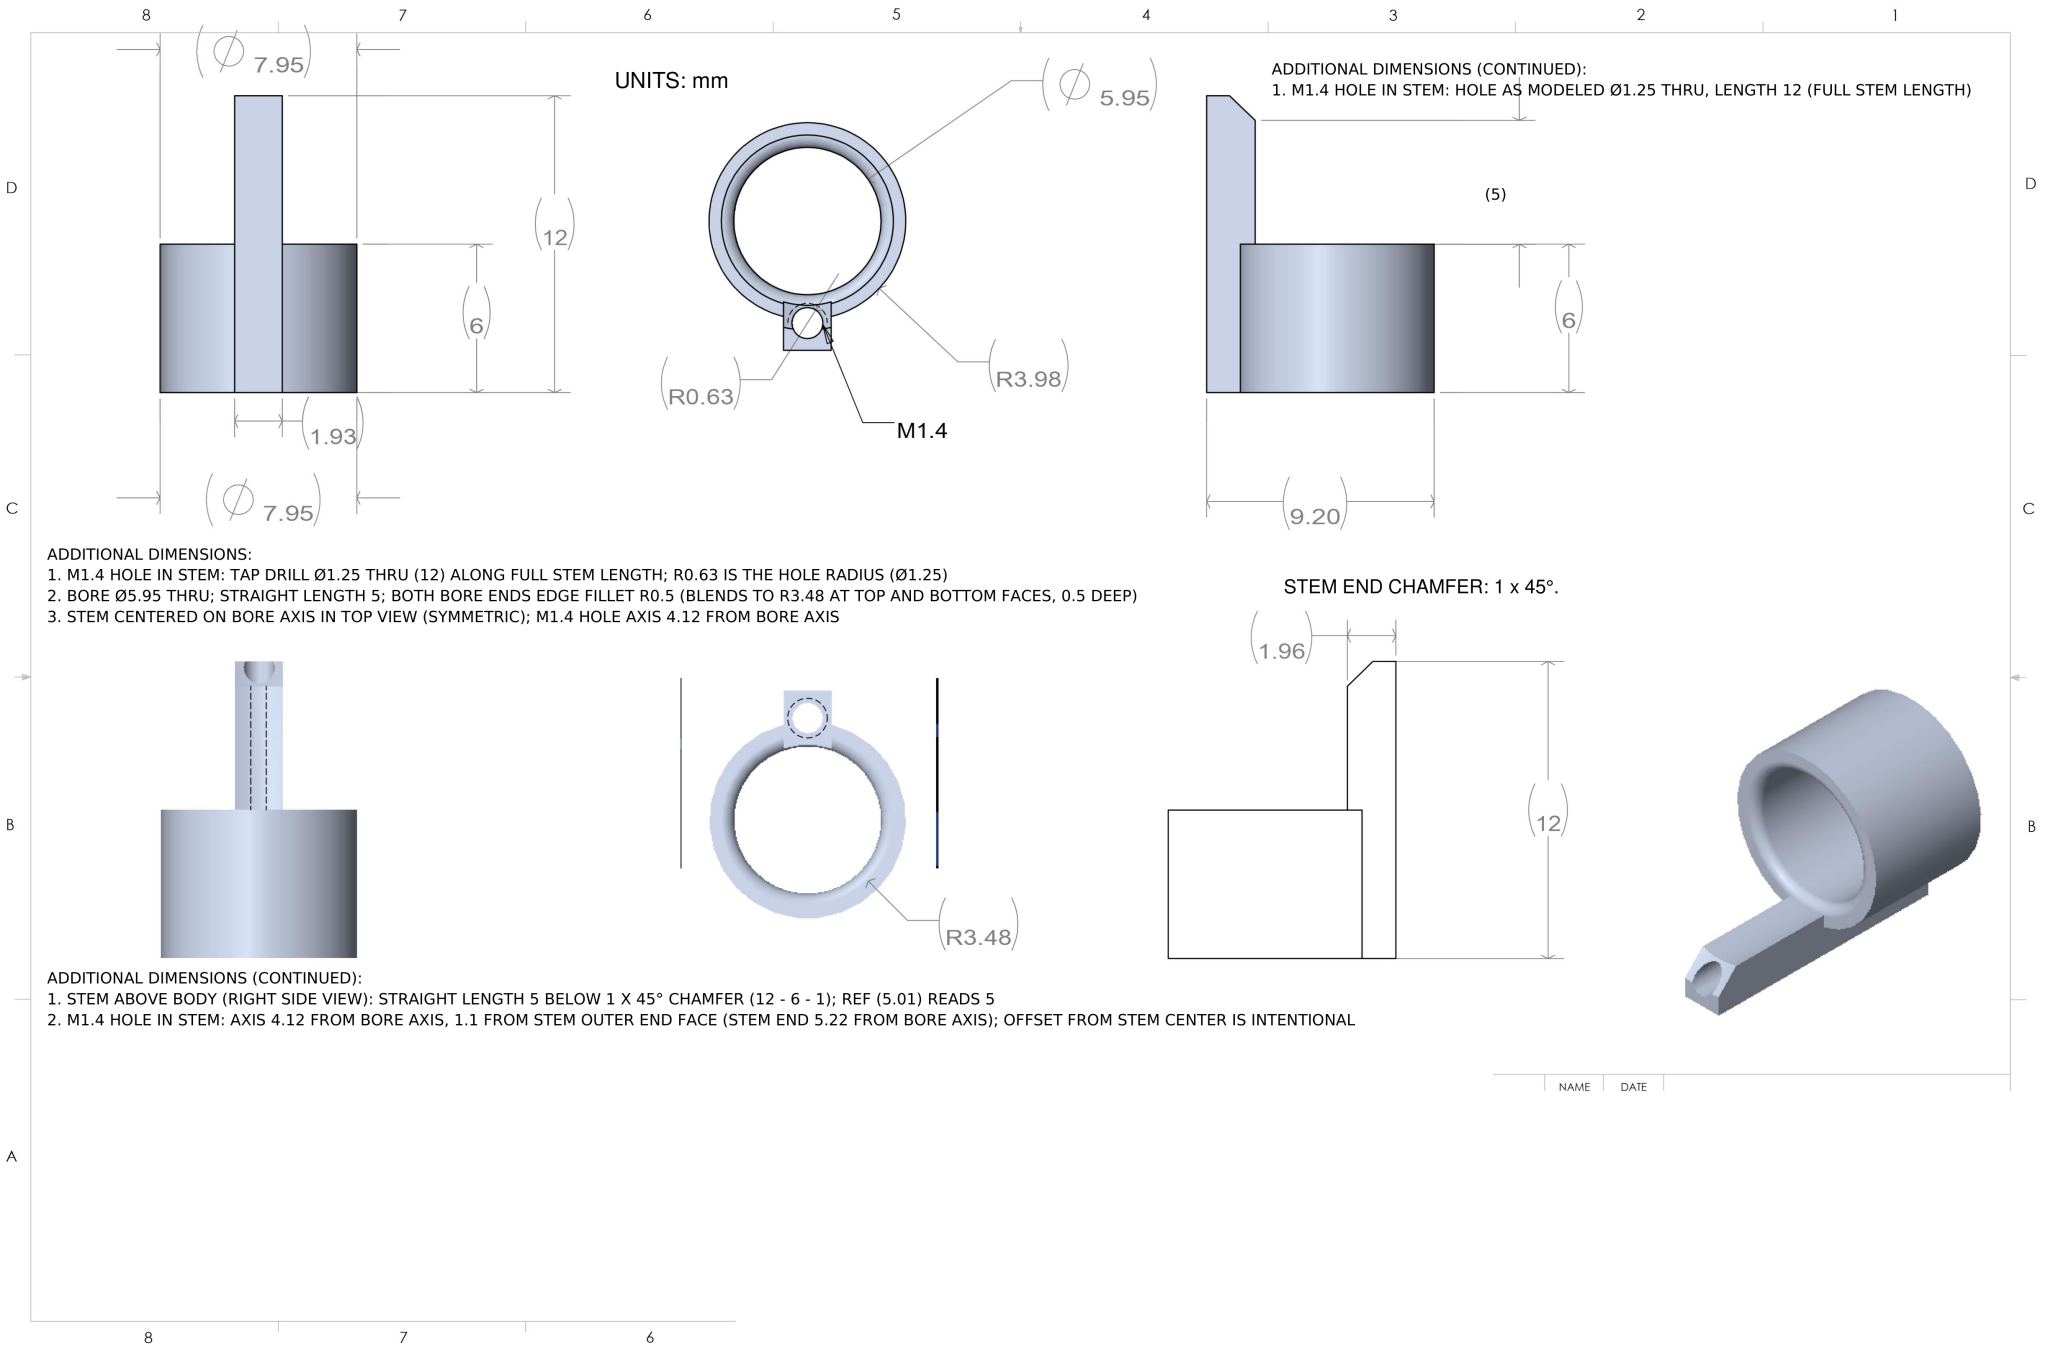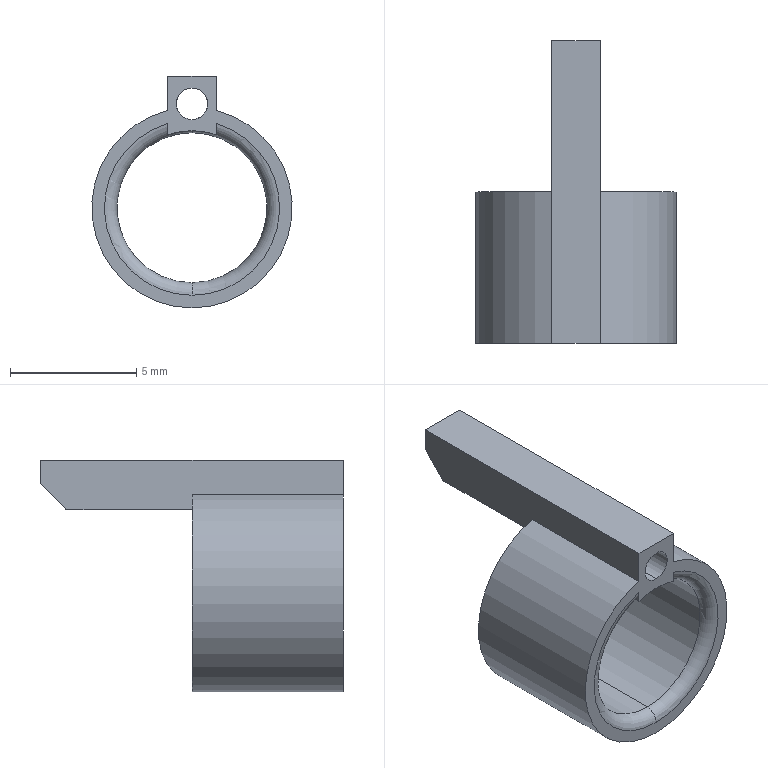Part | NX | mm | 1 solid | 22 faces | box 7.95 x 12 x 9.2 mm | volume 150 mm3 | cylinder 8 | plane 8 | torus 4 | cone 2 | commonest cylinder face diameters 1.25 x2 6.1 x2 5.95 x2 7.95 x1 6.8 x1
STEP:
#1=CARTESIAN_POINT('',(-0.5769,74.,8.153));
#2=VERTEX_POINT('',#1);
#3=CARTESIAN_POINT('',(0.,74.,8.538));
#4=VERTEX_POINT('',#3);
#5=CARTESIAN_POINT('',(0.,74.,7.913));
#6=DIRECTION('',(0.,1.,0.));
#7=DIRECTION('',(0.,0.,1.));
#8=AXIS2_PLACEMENT_3D('',#5,#6,#7);
#9=CIRCLE('',#8,0.625);
#10=EDGE_CURVE('',#2,#4,#9,.T.);
#11=ORIENTED_EDGE('',*,*,#10,.T.);
#12=CARTESIAN_POINT('',(0.,62.,8.538));
#13=VERTEX_POINT('',#12);
#14=CARTESIAN_POINT('',(0.,62.,8.538));
#15=DIRECTION('',(0.,-1.,0.));
#16=VECTOR('',#15,1000.);
#17=LINE('',#14,#16);
#18=EDGE_CURVE('',#4,#13,#17,.T.);
#19=ORIENTED_EDGE('',*,*,#18,.T.);
#20=CARTESIAN_POINT('',(0.,62.,7.288));
#21=VERTEX_POINT('',#20);
#22=CARTESIAN_POINT('',(0.,62.,7.913));
#23=DIRECTION('',(0.,-1.,0.));
#24=DIRECTION('',(0.,0.,-1.));
#25=AXIS2_PLACEMENT_3D('',#22,#23,#24);
#26=CIRCLE('',#25,0.625);
#27=EDGE_CURVE('',#13,#21,#26,.T.);
#28=ORIENTED_EDGE('',*,*,#27,.T.);
#29=CARTESIAN_POINT('',(-0.,73.097,7.288));
#30=VERTEX_POINT('',#29);
#31=CARTESIAN_POINT('',(0.,62.,7.288));
#32=DIRECTION('',(0.,-1.,0.));
#33=VECTOR('',#32,1000.);
#34=LINE('',#31,#33);
#35=EDGE_CURVE('',#30,#21,#34,.T.);
#36=ORIENTED_EDGE('',*,*,#35,.F.);
#37=CARTESIAN_POINT('',(-0.,73.097,7.288));
#38=CARTESIAN_POINT('',(-0.1316,73.097,7.288));
#39=CARTESIAN_POINT('',(-0.2545,73.149,7.332));
#40=CARTESIAN_POINT('',(-0.437,73.287,7.453));
#41=CARTESIAN_POINT('',(-0.5029,73.372,7.53));
#42=CARTESIAN_POINT('',(-0.5938,73.55,7.696));
#43=CARTESIAN_POINT('',(-0.6186,73.641,7.785));
#44=CARTESIAN_POINT('',(-0.6293,73.824,7.968));
#45=CARTESIAN_POINT('',(-0.6149,73.915,8.062));
#46=CARTESIAN_POINT('',(-0.5769,74.,8.153));
#47=B_SPLINE_CURVE_WITH_KNOTS('',3,(#37,#38,#39,#40,#41,#42,#43,#44,#45,#46),.UNSPECIFIED.,.F.,.F.,(4,2,2,2,4),(0.001551,0.001939,0.002327,0.002715,0.003103),.UNSPECIFIED.);
#48=EDGE_CURVE('',#30,#2,#47,.T.);
#49=ORIENTED_EDGE('',*,*,#48,.T.);
#50=EDGE_LOOP('',(#11,#19,#28,#36,#49));
#51=FACE_OUTER_BOUND('',#50,.T.);
#52=CARTESIAN_POINT('',(0.,62.,7.913));
#53=DIRECTION('',(0.,-1.,0.));
#54=DIRECTION('',(0.,0.,-1.));
#55=AXIS2_PLACEMENT_3D('',#52,#53,#54);
#56=CYLINDRICAL_SURFACE('',#55,0.625);
#57=ADVANCED_FACE('',(#51),#56,.F.);
#58=CARTESIAN_POINT('',(0.,73.,7.191));
#59=VERTEX_POINT('',#58);
#60=CARTESIAN_POINT('',(0.963,73.,7.052));
#61=VERTEX_POINT('',#60);
#62=CARTESIAN_POINT('',(0.,73.,3.791));
#63=DIRECTION('',(0.,1.,0.));
#64=DIRECTION('',(0.,0.,1.));
#65=AXIS2_PLACEMENT_3D('',#62,#63,#64);
#66=CIRCLE('',#65,3.4);
#67=EDGE_CURVE('',#59,#61,#66,.T.);
#68=ORIENTED_EDGE('',*,*,#67,.F.);
#69=CARTESIAN_POINT('',(0.,74.,8.191));
#70=DIRECTION('',(0.,0.7071,0.7071));
#71=VECTOR('',#70,1000.);
#72=LINE('',#69,#71);
#73=EDGE_CURVE('',#59,#30,#72,.T.);
#74=ORIENTED_EDGE('',*,*,#73,.T.);
#75=CARTESIAN_POINT('',(0.5769,74.,8.153));
#76=VERTEX_POINT('',#75);
#77=CARTESIAN_POINT('',(0.5769,74.,8.153));
#78=CARTESIAN_POINT('',(0.6149,73.915,8.062));
#79=CARTESIAN_POINT('',(0.6293,73.824,7.968));
#80=CARTESIAN_POINT('',(0.6186,73.642,7.785));
#81=CARTESIAN_POINT('',(0.5936,73.549,7.696));
#82=CARTESIAN_POINT('',(0.5029,73.372,7.53));
#83=CARTESIAN_POINT('',(0.4369,73.287,7.453));
#84=CARTESIAN_POINT('',(0.2542,73.148,7.332));
#85=CARTESIAN_POINT('',(0.1316,73.097,7.288));
#86=CARTESIAN_POINT('',(-0.,73.097,7.288));
#87=B_SPLINE_CURVE_WITH_KNOTS('',3,(#77,#78,#79,#80,#81,#82,#83,#84,#85,#86),.UNSPECIFIED.,.F.,.F.,(4,2,2,2,4),(0.0000003,0.0003881,0.0007758,0.001164,0.001551),.UNSPECIFIED.);
#88=EDGE_CURVE('',#76,#30,#87,.T.);
#89=ORIENTED_EDGE('',*,*,#88,.F.);
#90=CARTESIAN_POINT('',(0.963,74.,8.085));
#91=VERTEX_POINT('',#90);
#92=CARTESIAN_POINT('',(0.,74.,3.791));
#93=DIRECTION('',(0.,-1.,0.));
#94=DIRECTION('',(-0.,0.,1.));
#95=AXIS2_PLACEMENT_3D('',#92,#93,#94);
#96=CIRCLE('',#95,4.4);
#97=EDGE_CURVE('',#91,#76,#96,.T.);
#98=ORIENTED_EDGE('',*,*,#97,.F.);
#99=CARTESIAN_POINT('',(0.963,73.,7.052));
#100=CARTESIAN_POINT('',(0.963,73.332,7.398));
#101=CARTESIAN_POINT('',(0.963,73.665,7.742));
#102=CARTESIAN_POINT('',(0.963,74.,8.085));
#103=B_SPLINE_CURVE_WITH_KNOTS('',3,(#99,#100,#101,#102),.UNSPECIFIED.,.F.,.F.,(4,4),(0.,0.001437),.UNSPECIFIED.);
#104=EDGE_CURVE('',#61,#91,#103,.T.);
#105=ORIENTED_EDGE('',*,*,#104,.F.);
#106=EDGE_LOOP('',(#68,#74,#89,#98,#105));
#107=FACE_OUTER_BOUND('',#106,.T.);
#108=CARTESIAN_POINT('',(0.,74.,3.791));
#109=DIRECTION('',(0.,1.,0.));
#110=DIRECTION('',(0.,0.,1.));
#111=AXIS2_PLACEMENT_3D('',#108,#109,#110);
#112=CONICAL_SURFACE('',#111,4.4,0.7854);
#113=ADVANCED_FACE('',(#107),#112,.F.);
#114=CARTESIAN_POINT('',(0.,68.,0.3163));
#115=VERTEX_POINT('',#114);
#116=CARTESIAN_POINT('',(0.963,68.,7.13));
#117=VERTEX_POINT('',#116);
#118=CARTESIAN_POINT('',(0.,68.,3.791));
#119=DIRECTION('',(0.,-1.,0.));
#120=DIRECTION('',(0.,0.,1.));
#121=AXIS2_PLACEMENT_3D('',#118,#119,#120);
#122=CIRCLE('',#121,3.475);
#123=EDGE_CURVE('',#115,#117,#122,.T.);
#124=ORIENTED_EDGE('',*,*,#123,.F.);
#125=CARTESIAN_POINT('',(0.,67.5,0.8163));
#126=VERTEX_POINT('',#125);
#127=CARTESIAN_POINT('',(0.,67.5,0.3163));
#128=DIRECTION('',(1.,0.,0.));
#129=DIRECTION('',(0.,0.,-1.));
#130=AXIS2_PLACEMENT_3D('',#127,#128,#129);
#131=CIRCLE('',#130,0.5);
#132=EDGE_CURVE('',#115,#126,#131,.T.);
#133=ORIENTED_EDGE('',*,*,#132,.T.);
#134=CARTESIAN_POINT('',(0.,67.5,6.766));
#135=VERTEX_POINT('',#134);
#136=CARTESIAN_POINT('',(0.,67.5,3.791));
#137=DIRECTION('',(0.,1.,0.));
#138=DIRECTION('',(0.,0.,1.));
#139=AXIS2_PLACEMENT_3D('',#136,#137,#138);
#140=CIRCLE('',#139,2.975);
#141=EDGE_CURVE('',#135,#126,#140,.T.);
#142=ORIENTED_EDGE('',*,*,#141,.F.);
#143=CARTESIAN_POINT('',(0.,67.994,7.191));
#144=VERTEX_POINT('',#143);
#145=CARTESIAN_POINT('',(0.,67.5,7.266));
#146=DIRECTION('',(-1.,0.,0.));
#147=DIRECTION('',(0.,0.,1.));
#148=AXIS2_PLACEMENT_3D('',#145,#146,#147);
#149=CIRCLE('',#148,0.5);
#150=EDGE_CURVE('',#144,#135,#149,.T.);
#151=ORIENTED_EDGE('',*,*,#150,.F.);
#152=CARTESIAN_POINT('',(0.963,67.994,7.052));
#153=VERTEX_POINT('',#152);
#154=CARTESIAN_POINT('',(0.,67.994,3.791));
#155=DIRECTION('',(0.,-1.,0.));
#156=DIRECTION('',(0.,0.,-1.));
#157=AXIS2_PLACEMENT_3D('',#154,#155,#156);
#158=CIRCLE('',#157,3.4);
#159=EDGE_CURVE('',#153,#144,#158,.T.);
#160=ORIENTED_EDGE('',*,*,#159,.F.);
#161=CARTESIAN_POINT('',(0.963,67.994,7.052));
#162=CARTESIAN_POINT('',(0.963,67.996,7.065));
#163=CARTESIAN_POINT('',(0.963,67.999,7.091));
#164=CARTESIAN_POINT('',(0.963,68.,7.117));
#165=CARTESIAN_POINT('',(0.963,68.,7.13));
#166=B_SPLINE_CURVE_WITH_KNOTS('',3,(#161,#162,#163,#164,#165),.UNSPECIFIED.,.F.,.F.,(4,1,4),(0.0003591,0.0003981,0.0004371),.UNSPECIFIED.);
#167=EDGE_CURVE('',#153,#117,#166,.T.);
#168=ORIENTED_EDGE('',*,*,#167,.T.);
#169=EDGE_LOOP('',(#124,#133,#142,#151,#160,#168));
#170=FACE_OUTER_BOUND('',#169,.T.);
#171=CARTESIAN_POINT('',(0.,67.5,3.791));
#172=DIRECTION('',(0.,1.,0.));
#173=DIRECTION('',(0.,0.,1.));
#174=AXIS2_PLACEMENT_3D('',#171,#172,#173);
#175=TOROIDAL_SURFACE('',#174,3.475,0.5);
#176=ADVANCED_FACE('',(#170),#175,.T.);
#177=CARTESIAN_POINT('',(0.,62.,6.841));
#178=VERTEX_POINT('',#177);
#179=CARTESIAN_POINT('',(0.963,62.,6.685));
#180=VERTEX_POINT('',#179);
#181=CARTESIAN_POINT('',(0.,62.,3.791));
#182=DIRECTION('',(0.,1.,-0.));
#183=DIRECTION('',(0.,0.,-1.));
#184=AXIS2_PLACEMENT_3D('',#181,#182,#183);
#185=CIRCLE('',#184,3.05);
#186=EDGE_CURVE('',#178,#180,#185,.T.);
#187=ORIENTED_EDGE('',*,*,#186,.F.);
#188=CARTESIAN_POINT('',(0.,62.237,6.841));
#189=VERTEX_POINT('',#188);
#190=CARTESIAN_POINT('',(0.,10.423,6.841));
#191=DIRECTION('',(0.,1.,0.));
#192=VECTOR('',#191,1000.);
#193=LINE('',#190,#192);
#194=EDGE_CURVE('',#178,#189,#193,.T.);
#195=ORIENTED_EDGE('',*,*,#194,.T.);
#196=CARTESIAN_POINT('',(0.963,62.237,6.685));
#197=VERTEX_POINT('',#196);
#198=CARTESIAN_POINT('',(0.,62.237,3.791));
#199=DIRECTION('',(0.,-1.,0.));
#200=DIRECTION('',(0.,0.,1.));
#201=AXIS2_PLACEMENT_3D('',#198,#199,#200);
#202=CIRCLE('',#201,3.05);
#203=EDGE_CURVE('',#197,#189,#202,.T.);
#204=ORIENTED_EDGE('',*,*,#203,.F.);
#205=CARTESIAN_POINT('',(0.963,10.423,6.685));
#206=DIRECTION('',(0.,1.,0.));
#207=VECTOR('',#206,1000.);
#208=LINE('',#205,#207);
#209=EDGE_CURVE('',#180,#197,#208,.T.);
#210=ORIENTED_EDGE('',*,*,#209,.F.);
#211=EDGE_LOOP('',(#187,#195,#204,#210));
#212=FACE_OUTER_BOUND('',#211,.T.);
#213=CARTESIAN_POINT('',(0.,10.423,3.791));
#214=DIRECTION('',(0.,1.,0.));
#215=DIRECTION('',(0.,0.,1.));
#216=AXIS2_PLACEMENT_3D('',#213,#214,#215);
#217=CYLINDRICAL_SURFACE('',#216,3.05);
#218=ADVANCED_FACE('',(#212),#217,.F.);
#219=CARTESIAN_POINT('',(0.,62.5,0.8163));
#220=VERTEX_POINT('',#219);
#221=CARTESIAN_POINT('',(0.,62.5,6.766));
#222=VERTEX_POINT('',#221);
#223=CARTESIAN_POINT('',(0.,62.5,3.791));
#224=DIRECTION('',(0.,-1.,0.));
#225=DIRECTION('',(0.,0.,1.));
#226=AXIS2_PLACEMENT_3D('',#223,#224,#225);
#227=CIRCLE('',#226,2.975);
#228=EDGE_CURVE('',#220,#222,#227,.T.);
#229=ORIENTED_EDGE('',*,*,#228,.F.);
#230=CARTESIAN_POINT('',(0.,62.,0.3163));
#231=VERTEX_POINT('',#230);
#232=CARTESIAN_POINT('',(0.,62.5,0.3163));
#233=DIRECTION('',(1.,0.,0.));
#234=DIRECTION('',(0.,0.,-1.));
#235=AXIS2_PLACEMENT_3D('',#232,#233,#234);
#236=CIRCLE('',#235,0.5);
#237=EDGE_CURVE('',#220,#231,#236,.T.);
#238=ORIENTED_EDGE('',*,*,#237,.T.);
#239=CARTESIAN_POINT('',(0.963,62.,7.13));
#240=VERTEX_POINT('',#239);
#241=CARTESIAN_POINT('',(0.,62.,3.791));
#242=DIRECTION('',(0.,1.,0.));
#243=DIRECTION('',(0.,0.,1.));
#244=AXIS2_PLACEMENT_3D('',#241,#242,#243);
#245=CIRCLE('',#244,3.475);
#246=EDGE_CURVE('',#240,#231,#245,.T.);
#247=ORIENTED_EDGE('',*,*,#246,.F.);
#248=CARTESIAN_POINT('',(0.963,62.,7.13));
#249=CARTESIAN_POINT('',(0.963,62.,7.043));
#250=CARTESIAN_POINT('',(0.963,62.021,6.956));
#251=CARTESIAN_POINT('',(0.963,62.103,6.8));
#252=CARTESIAN_POINT('',(0.963,62.163,6.734));
#253=CARTESIAN_POINT('',(0.963,62.237,6.685));
#254=B_SPLINE_CURVE_WITH_KNOTS('',3,(#248,#249,#250,#251,#252,#253),.UNSPECIFIED.,.F.,.F.,(4,2,4),(0.002836,0.003097,0.003358),.UNSPECIFIED.);
#255=EDGE_CURVE('',#240,#197,#254,.T.);
#256=ORIENTED_EDGE('',*,*,#255,.T.);
#257=ORIENTED_EDGE('',*,*,#203,.T.);
#258=CARTESIAN_POINT('',(0.,62.5,7.266));
#259=DIRECTION('',(-1.,0.,0.));
#260=DIRECTION('',(0.,0.,1.));
#261=AXIS2_PLACEMENT_3D('',#258,#259,#260);
#262=CIRCLE('',#261,0.5);
#263=EDGE_CURVE('',#222,#189,#262,.T.);
#264=ORIENTED_EDGE('',*,*,#263,.F.);
#265=EDGE_LOOP('',(#229,#238,#247,#256,#257,#264));
#266=FACE_OUTER_BOUND('',#265,.T.);
#267=CARTESIAN_POINT('',(0.,62.5,3.791));
#268=DIRECTION('',(0.,1.,0.));
#269=DIRECTION('',(0.,0.,1.));
#270=AXIS2_PLACEMENT_3D('',#267,#268,#269);
#271=TOROIDAL_SURFACE('',#270,3.475,0.5);
#272=ADVANCED_FACE('',(#266),#271,.T.);
#273=CARTESIAN_POINT('',(0.,62.5,3.791));
#274=DIRECTION('',(0.,-1.,0.));
#275=DIRECTION('',(0.,0.,1.));
#276=AXIS2_PLACEMENT_3D('',#273,#274,#275);
#277=CIRCLE('',#276,2.975);
#278=EDGE_CURVE('',#222,#220,#277,.T.);
#279=ORIENTED_EDGE('',*,*,#278,.T.);
#280=CARTESIAN_POINT('',(0.,62.,0.8163));
#281=DIRECTION('',(0.,1.,0.));
#282=VECTOR('',#281,1000.);
#283=LINE('',#280,#282);
#284=EDGE_CURVE('',#220,#126,#283,.T.);
#285=ORIENTED_EDGE('',*,*,#284,.T.);
#286=CARTESIAN_POINT('',(0.,67.5,3.791));
#287=DIRECTION('',(0.,1.,0.));
#288=DIRECTION('',(0.,0.,1.));
#289=AXIS2_PLACEMENT_3D('',#286,#287,#288);
#290=CIRCLE('',#289,2.975);
#291=EDGE_CURVE('',#126,#135,#290,.T.);
#292=ORIENTED_EDGE('',*,*,#291,.T.);
#293=CARTESIAN_POINT('',(0.,62.,6.766));
#294=DIRECTION('',(0.,1.,0.));
#295=VECTOR('',#294,1000.);
#296=LINE('',#293,#295);
#297=EDGE_CURVE('',#222,#135,#296,.T.);
#298=ORIENTED_EDGE('',*,*,#297,.F.);
#299=EDGE_LOOP('',(#279,#285,#292,#298));
#300=FACE_OUTER_BOUND('',#299,.T.);
#301=CARTESIAN_POINT('',(0.,62.,3.791));
#302=DIRECTION('',(0.,1.,0.));
#303=DIRECTION('',(0.,0.,1.));
#304=AXIS2_PLACEMENT_3D('',#301,#302,#303);
#305=CYLINDRICAL_SURFACE('',#304,2.975);
#306=ADVANCED_FACE('',(#300),#305,.F.);
#307=ORIENTED_EDGE('',*,*,#284,.F.);
#308=ORIENTED_EDGE('',*,*,#228,.T.);
#309=ORIENTED_EDGE('',*,*,#297,.T.);
#310=ORIENTED_EDGE('',*,*,#141,.T.);
#311=EDGE_LOOP('',(#307,#308,#309,#310));
#312=FACE_OUTER_BOUND('',#311,.T.);
#313=CARTESIAN_POINT('',(0.,62.,3.791));
#314=DIRECTION('',(0.,1.,0.));
#315=DIRECTION('',(0.,0.,1.));
#316=AXIS2_PLACEMENT_3D('',#313,#314,#315);
#317=CYLINDRICAL_SURFACE('',#316,2.975);
#318=ADVANCED_FACE('',(#312),#317,.F.);
#319=CARTESIAN_POINT('',(0.963,62.,6.38));
#320=DIRECTION('',(0.,0.,1.));
#321=VECTOR('',#320,1000.);
#322=LINE('',#319,#321);
#323=EDGE_CURVE('',#180,#240,#322,.T.);
#324=ORIENTED_EDGE('',*,*,#323,.F.);
#325=ORIENTED_EDGE('',*,*,#209,.T.);
#326=ORIENTED_EDGE('',*,*,#255,.F.);
#327=EDGE_LOOP('',(#324,#325,#326));
#328=FACE_OUTER_BOUND('',#327,.T.);
#329=CARTESIAN_POINT('',(0.963,74.,6.38));
#330=DIRECTION('',(-1.,0.,0.));
#331=DIRECTION('',(0.,0.,1.));
#332=AXIS2_PLACEMENT_3D('',#329,#330,#331);
#333=PLANE('',#332);
#334=ADVANCED_FACE('',(#328),#333,.F.);
#335=ORIENTED_EDGE('',*,*,#237,.F.);
#336=ORIENTED_EDGE('',*,*,#278,.F.);
#337=ORIENTED_EDGE('',*,*,#263,.T.);
#338=CARTESIAN_POINT('',(-0.963,62.237,6.685));
#339=VERTEX_POINT('',#338);
#340=CARTESIAN_POINT('',(0.,62.237,3.791));
#341=DIRECTION('',(0.,-1.,0.));
#342=DIRECTION('',(0.,0.,1.));
#343=AXIS2_PLACEMENT_3D('',#340,#341,#342);
#344=CIRCLE('',#343,3.05);
#345=EDGE_CURVE('',#189,#339,#344,.T.);
#346=ORIENTED_EDGE('',*,*,#345,.T.);
#347=CARTESIAN_POINT('',(-0.963,62.,7.13));
#348=VERTEX_POINT('',#347);
#349=CARTESIAN_POINT('',(-0.963,62.237,6.685));
#350=CARTESIAN_POINT('',(-0.963,62.164,6.733));
#351=CARTESIAN_POINT('',(-0.963,62.103,6.801));
#352=CARTESIAN_POINT('',(-0.963,62.022,6.955));
#353=CARTESIAN_POINT('',(-0.963,62.,7.042));
#354=CARTESIAN_POINT('',(-0.963,62.,7.13));
#355=B_SPLINE_CURVE_WITH_KNOTS('',3,(#349,#350,#351,#352,#353,#354),.UNSPECIFIED.,.F.,.F.,(4,2,4),(0.003024,0.003285,0.003546),.UNSPECIFIED.);
#356=EDGE_CURVE('',#339,#348,#355,.T.);
#357=ORIENTED_EDGE('',*,*,#356,.T.);
#358=CARTESIAN_POINT('',(0.,62.,3.791));
#359=DIRECTION('',(0.,1.,0.));
#360=DIRECTION('',(0.,0.,1.));
#361=AXIS2_PLACEMENT_3D('',#358,#359,#360);
#362=CIRCLE('',#361,3.475);
#363=EDGE_CURVE('',#231,#348,#362,.T.);
#364=ORIENTED_EDGE('',*,*,#363,.F.);
#365=EDGE_LOOP('',(#335,#336,#337,#346,#357,#364));
#366=FACE_OUTER_BOUND('',#365,.T.);
#367=CARTESIAN_POINT('',(0.,62.5,3.791));
#368=DIRECTION('',(0.,1.,0.));
#369=DIRECTION('',(0.,0.,1.));
#370=AXIS2_PLACEMENT_3D('',#367,#368,#369);
#371=TOROIDAL_SURFACE('',#370,3.475,0.5);
#372=ADVANCED_FACE('',(#366),#371,.T.);
#373=CARTESIAN_POINT('',(-0.963,62.,6.685));
#374=VERTEX_POINT('',#373);
#375=CARTESIAN_POINT('',(-0.963,62.,6.38));
#376=DIRECTION('',(-0.,-0.,-1.));
#377=VECTOR('',#376,1000.);
#378=LINE('',#375,#377);
#379=EDGE_CURVE('',#348,#374,#378,.T.);
#380=ORIENTED_EDGE('',*,*,#379,.F.);
#381=ORIENTED_EDGE('',*,*,#356,.F.);
#382=CARTESIAN_POINT('',(-0.963,10.423,6.685));
#383=DIRECTION('',(0.,-1.,0.));
#384=VECTOR('',#383,1000.);
#385=LINE('',#382,#384);
#386=EDGE_CURVE('',#339,#374,#385,.T.);
#387=ORIENTED_EDGE('',*,*,#386,.T.);
#388=EDGE_LOOP('',(#380,#381,#387));
#389=FACE_OUTER_BOUND('',#388,.T.);
#390=CARTESIAN_POINT('',(-0.963,74.,6.38));
#391=DIRECTION('',(1.,0.,-0.));
#392=DIRECTION('',(-0.,0.,-1.));
#393=AXIS2_PLACEMENT_3D('',#390,#391,#392);
#394=PLANE('',#393);
#395=ADVANCED_FACE('',(#389),#394,.F.);
#396=ORIENTED_EDGE('',*,*,#194,.F.);
#397=CARTESIAN_POINT('',(0.,62.,3.791));
#398=DIRECTION('',(0.,1.,-0.));
#399=DIRECTION('',(0.,0.,-1.));
#400=AXIS2_PLACEMENT_3D('',#397,#398,#399);
#401=CIRCLE('',#400,3.05);
#402=EDGE_CURVE('',#374,#178,#401,.T.);
#403=ORIENTED_EDGE('',*,*,#402,.F.);
#404=ORIENTED_EDGE('',*,*,#386,.F.);
#405=ORIENTED_EDGE('',*,*,#345,.F.);
#406=EDGE_LOOP('',(#396,#403,#404,#405));
#407=FACE_OUTER_BOUND('',#406,.T.);
#408=CARTESIAN_POINT('',(0.,10.423,3.791));
#409=DIRECTION('',(0.,1.,0.));
#410=DIRECTION('',(0.,0.,1.));
#411=AXIS2_PLACEMENT_3D('',#408,#409,#410);
#412=CYLINDRICAL_SURFACE('',#411,3.05);
#413=ADVANCED_FACE('',(#407),#412,.F.);
#414=CARTESIAN_POINT('',(0.963,68.,7.648));
#415=VERTEX_POINT('',#414);
#416=CARTESIAN_POINT('',(-0.963,68.,7.648));
#417=VERTEX_POINT('',#416);
#418=CARTESIAN_POINT('',(0.,68.,3.791));
#419=DIRECTION('',(0.,1.,0.));
#420=DIRECTION('',(1.,0.,0.));
#421=AXIS2_PLACEMENT_3D('',#418,#419,#420);
#422=CIRCLE('',#421,3.975);
#423=EDGE_CURVE('',#415,#417,#422,.T.);
#424=ORIENTED_EDGE('',*,*,#423,.F.);
#425=CARTESIAN_POINT('',(0.963,62.,7.648));
#426=VERTEX_POINT('',#425);
#427=CARTESIAN_POINT('',(0.963,62.,7.648));
#428=DIRECTION('',(0.,-1.,0.));
#429=VECTOR('',#428,1000.);
#430=LINE('',#427,#429);
#431=EDGE_CURVE('',#415,#426,#430,.T.);
#432=ORIENTED_EDGE('',*,*,#431,.T.);
#433=CARTESIAN_POINT('',(-0.963,62.,7.648));
#434=VERTEX_POINT('',#433);
#435=CARTESIAN_POINT('',(0.,62.,3.791));
#436=DIRECTION('',(0.,1.,0.));
#437=DIRECTION('',(1.,0.,0.));
#438=AXIS2_PLACEMENT_3D('',#435,#436,#437);
#439=CIRCLE('',#438,3.975);
#440=EDGE_CURVE('',#426,#434,#439,.T.);
#441=ORIENTED_EDGE('',*,*,#440,.T.);
#442=CARTESIAN_POINT('',(-0.963,62.,7.648));
#443=DIRECTION('',(0.,1.,0.));
#444=VECTOR('',#443,1000.);
#445=LINE('',#442,#444);
#446=EDGE_CURVE('',#434,#417,#445,.T.);
#447=ORIENTED_EDGE('',*,*,#446,.T.);
#448=EDGE_LOOP('',(#424,#432,#441,#447));
#449=FACE_OUTER_BOUND('',#448,.T.);
#450=CARTESIAN_POINT('',(0.,62.,3.791));
#451=DIRECTION('',(0.,1.,0.));
#452=DIRECTION('',(0.,0.,1.));
#453=AXIS2_PLACEMENT_3D('',#450,#451,#452);
#454=CYLINDRICAL_SURFACE('',#453,3.975);
#455=ADVANCED_FACE('',(#449),#454,.T.);
#456=CARTESIAN_POINT('',(-0.963,68.,7.13));
#457=VERTEX_POINT('',#456);
#458=CARTESIAN_POINT('',(0.,68.,3.791));
#459=DIRECTION('',(0.,-1.,0.));
#460=DIRECTION('',(0.,0.,1.));
#461=AXIS2_PLACEMENT_3D('',#458,#459,#460);
#462=CIRCLE('',#461,3.475);
#463=EDGE_CURVE('',#457,#115,#462,.T.);
#464=ORIENTED_EDGE('',*,*,#463,.T.);
#465=ORIENTED_EDGE('',*,*,#123,.T.);
#466=CARTESIAN_POINT('',(0.963,68.,3.791));
#467=DIRECTION('',(0.,0.,1.));
#468=VECTOR('',#467,1000.);
#469=LINE('',#466,#468);
#470=EDGE_CURVE('',#117,#415,#469,.T.);
#471=ORIENTED_EDGE('',*,*,#470,.T.);
#472=ORIENTED_EDGE('',*,*,#423,.T.);
#473=CARTESIAN_POINT('',(-0.963,68.,3.791));
#474=DIRECTION('',(-0.,0.,-1.));
#475=VECTOR('',#474,1000.);
#476=LINE('',#473,#475);
#477=EDGE_CURVE('',#417,#457,#476,.T.);
#478=ORIENTED_EDGE('',*,*,#477,.T.);
#479=EDGE_LOOP('',(#464,#465,#471,#472,#478));
#480=FACE_OUTER_BOUND('',#479,.T.);
#481=CARTESIAN_POINT('',(0.,68.,3.791));
#482=DIRECTION('',(0.,1.,0.));
#483=DIRECTION('',(0.,0.,1.));
#484=AXIS2_PLACEMENT_3D('',#481,#482,#483);
#485=PLANE('',#484);
#486=ADVANCED_FACE('',(#480),#485,.T.);
#487=ORIENTED_EDGE('',*,*,#132,.F.);
#488=ORIENTED_EDGE('',*,*,#463,.F.);
#489=CARTESIAN_POINT('',(-0.963,67.994,7.052));
#490=VERTEX_POINT('',#489);
#491=CARTESIAN_POINT('',(-0.963,68.,7.13));
#492=CARTESIAN_POINT('',(-0.963,68.,7.117));
#493=CARTESIAN_POINT('',(-0.963,67.999,7.091));
#494=CARTESIAN_POINT('',(-0.963,67.996,7.065));
#495=CARTESIAN_POINT('',(-0.963,67.994,7.052));
#496=B_SPLINE_CURVE_WITH_KNOTS('',3,(#491,#492,#493,#494,#495),.UNSPECIFIED.,.F.,.F.,(4,1,4),(0.002755,0.002795,0.002834),.UNSPECIFIED.);
#497=EDGE_CURVE('',#457,#490,#496,.T.);
#498=ORIENTED_EDGE('',*,*,#497,.T.);
#499=CARTESIAN_POINT('',(0.,67.994,3.791));
#500=DIRECTION('',(0.,-1.,0.));
#501=DIRECTION('',(0.,0.,-1.));
#502=AXIS2_PLACEMENT_3D('',#499,#500,#501);
#503=CIRCLE('',#502,3.4);
#504=EDGE_CURVE('',#144,#490,#503,.T.);
#505=ORIENTED_EDGE('',*,*,#504,.F.);
#506=ORIENTED_EDGE('',*,*,#150,.T.);
#507=ORIENTED_EDGE('',*,*,#291,.F.);
#508=EDGE_LOOP('',(#487,#488,#498,#505,#506,#507));
#509=FACE_OUTER_BOUND('',#508,.T.);
#510=CARTESIAN_POINT('',(0.,67.5,3.791));
#511=DIRECTION('',(0.,1.,0.));
#512=DIRECTION('',(0.,0.,1.));
#513=AXIS2_PLACEMENT_3D('',#510,#511,#512);
#514=TOROIDAL_SURFACE('',#513,3.475,0.5);
#515=ADVANCED_FACE('',(#509),#514,.T.);
#516=CARTESIAN_POINT('',(0.963,75.65,7.052));
#517=DIRECTION('',(0.,-1.,0.));
#518=VECTOR('',#517,1000.);
#519=LINE('',#516,#518);
#520=EDGE_CURVE('',#61,#153,#519,.T.);
#521=ORIENTED_EDGE('',*,*,#520,.T.);
#522=ORIENTED_EDGE('',*,*,#159,.T.);
#523=ORIENTED_EDGE('',*,*,#504,.T.);
#524=CARTESIAN_POINT('',(-0.963,73.,7.052));
#525=VERTEX_POINT('',#524);
#526=CARTESIAN_POINT('',(-0.963,75.65,7.052));
#527=DIRECTION('',(0.,1.,0.));
#528=VECTOR('',#527,1000.);
#529=LINE('',#526,#528);
#530=EDGE_CURVE('',#490,#525,#529,.T.);
#531=ORIENTED_EDGE('',*,*,#530,.T.);
#532=CARTESIAN_POINT('',(0.,73.,3.791));
#533=DIRECTION('',(0.,1.,0.));
#534=DIRECTION('',(0.,0.,1.));
#535=AXIS2_PLACEMENT_3D('',#532,#533,#534);
#536=CIRCLE('',#535,3.4);
#537=EDGE_CURVE('',#525,#59,#536,.T.);
#538=ORIENTED_EDGE('',*,*,#537,.T.);
#539=ORIENTED_EDGE('',*,*,#67,.T.);
#540=EDGE_LOOP('',(#521,#522,#523,#531,#538,#539));
#541=FACE_OUTER_BOUND('',#540,.T.);
#542=CARTESIAN_POINT('',(0.,75.65,3.791));
#543=DIRECTION('',(0.,-1.,0.));
#544=DIRECTION('',(0.,0.,-1.));
#545=AXIS2_PLACEMENT_3D('',#542,#543,#544);
#546=CYLINDRICAL_SURFACE('',#545,3.4);
#547=ADVANCED_FACE('',(#541),#546,.F.);
#548=ORIENTED_EDGE('',*,*,#73,.F.);
#549=ORIENTED_EDGE('',*,*,#537,.F.);
#550=CARTESIAN_POINT('',(-0.963,74.,8.085));
#551=VERTEX_POINT('',#550);
#552=CARTESIAN_POINT('',(-0.963,74.,8.085));
#553=CARTESIAN_POINT('',(-0.963,73.665,7.742));
#554=CARTESIAN_POINT('',(-0.963,73.332,7.398));
#555=CARTESIAN_POINT('',(-0.963,73.,7.052));
#556=B_SPLINE_CURVE_WITH_KNOTS('',3,(#552,#553,#554,#555),.UNSPECIFIED.,.F.,.F.,(4,4),(0.,0.001437),.UNSPECIFIED.);
#557=EDGE_CURVE('',#551,#525,#556,.T.);
#558=ORIENTED_EDGE('',*,*,#557,.F.);
#559=CARTESIAN_POINT('',(0.,74.,3.791));
#560=DIRECTION('',(0.,-1.,0.));
#561=DIRECTION('',(0.,0.,1.));
#562=AXIS2_PLACEMENT_3D('',#559,#560,#561);
#563=CIRCLE('',#562,4.4);
#564=EDGE_CURVE('',#2,#551,#563,.T.);
#565=ORIENTED_EDGE('',*,*,#564,.F.);
#566=ORIENTED_EDGE('',*,*,#48,.F.);
#567=EDGE_LOOP('',(#548,#549,#558,#565,#566));
#568=FACE_OUTER_BOUND('',#567,.T.);
#569=CARTESIAN_POINT('',(0.,74.,3.791));
#570=DIRECTION('',(0.,1.,0.));
#571=DIRECTION('',(0.,0.,1.));
#572=AXIS2_PLACEMENT_3D('',#569,#570,#571);
#573=CONICAL_SURFACE('',#572,4.4,0.7854);
#574=ADVANCED_FACE('',(#568),#573,.F.);
#575=CARTESIAN_POINT('',(0.963,62.,9.012));
#576=VERTEX_POINT('',#575);
#577=CARTESIAN_POINT('',(0.963,74.,9.012));
#578=VERTEX_POINT('',#577);
#579=CARTESIAN_POINT('',(0.963,74.,9.012));
#580=DIRECTION('',(0.,1.,0.));
#581=VECTOR('',#580,1000.);
#582=LINE('',#579,#581);
#583=EDGE_CURVE('',#576,#578,#582,.T.);
#584=ORIENTED_EDGE('',*,*,#583,.F.);
#585=CARTESIAN_POINT('',(0.963,62.,6.38));
#586=DIRECTION('',(0.,0.,1.));
#587=VECTOR('',#586,1000.);
#588=LINE('',#585,#587);
#589=EDGE_CURVE('',#426,#576,#588,.T.);
#590=ORIENTED_EDGE('',*,*,#589,.F.);
#591=ORIENTED_EDGE('',*,*,#431,.F.);
#592=ORIENTED_EDGE('',*,*,#470,.F.);
#593=ORIENTED_EDGE('',*,*,#167,.F.);
#594=ORIENTED_EDGE('',*,*,#520,.F.);
#595=ORIENTED_EDGE('',*,*,#104,.T.);
#596=CARTESIAN_POINT('',(0.963,74.,6.38));
#597=DIRECTION('',(0.,0.,-1.));
#598=VECTOR('',#597,1000.);
#599=LINE('',#596,#598);
#600=EDGE_CURVE('',#578,#91,#599,.T.);
#601=ORIENTED_EDGE('',*,*,#600,.F.);
#602=EDGE_LOOP('',(#584,#590,#591,#592,#593,#594,#595,#601));
#603=FACE_OUTER_BOUND('',#602,.T.);
#604=CARTESIAN_POINT('',(0.963,74.,6.38));
#605=DIRECTION('',(-1.,0.,0.));
#606=DIRECTION('',(0.,0.,1.));
#607=AXIS2_PLACEMENT_3D('',#604,#605,#606);
#608=PLANE('',#607);
#609=ADVANCED_FACE('',(#603),#608,.F.);
#610=CARTESIAN_POINT('',(-0.963,74.,9.012));
#611=VERTEX_POINT('',#610);
#612=CARTESIAN_POINT('',(-0.963,62.,9.012));
#613=VERTEX_POINT('',#612);
#614=CARTESIAN_POINT('',(-0.963,74.,9.012));
#615=DIRECTION('',(0.,-1.,0.));
#616=VECTOR('',#615,1000.);
#617=LINE('',#614,#616);
#618=EDGE_CURVE('',#611,#613,#617,.T.);
#619=ORIENTED_EDGE('',*,*,#618,.F.);
#620=CARTESIAN_POINT('',(-0.963,74.,6.38));
#621=DIRECTION('',(0.,0.,1.));
#622=VECTOR('',#621,1000.);
#623=LINE('',#620,#622);
#624=EDGE_CURVE('',#551,#611,#623,.T.);
#625=ORIENTED_EDGE('',*,*,#624,.F.);
#626=ORIENTED_EDGE('',*,*,#557,.T.);
#627=ORIENTED_EDGE('',*,*,#530,.F.);
#628=ORIENTED_EDGE('',*,*,#497,.F.);
#629=ORIENTED_EDGE('',*,*,#477,.F.);
#630=ORIENTED_EDGE('',*,*,#446,.F.);
#631=CARTESIAN_POINT('',(-0.963,62.,6.38));
#632=DIRECTION('',(-0.,-0.,-1.));
#633=VECTOR('',#632,1000.);
#634=LINE('',#631,#633);
#635=EDGE_CURVE('',#613,#434,#634,.T.);
#636=ORIENTED_EDGE('',*,*,#635,.F.);
#637=EDGE_LOOP('',(#619,#625,#626,#627,#628,#629,#630,#636));
#638=FACE_OUTER_BOUND('',#637,.T.);
#639=CARTESIAN_POINT('',(-0.963,74.,6.38));
#640=DIRECTION('',(1.,0.,-0.));
#641=DIRECTION('',(-0.,0.,-1.));
#642=AXIS2_PLACEMENT_3D('',#639,#640,#641);
#643=PLANE('',#642);
#644=ADVANCED_FACE('',(#638),#643,.F.);
#645=ORIENTED_EDGE('',*,*,#10,.F.);
#646=ORIENTED_EDGE('',*,*,#564,.T.);
#647=ORIENTED_EDGE('',*,*,#624,.T.);
#648=CARTESIAN_POINT('',(0.,74.,9.012));
#649=DIRECTION('',(1.,0.,0.));
#650=VECTOR('',#649,1000.);
#651=LINE('',#648,#650);
#652=EDGE_CURVE('',#611,#578,#651,.T.);
#653=ORIENTED_EDGE('',*,*,#652,.T.);
#654=ORIENTED_EDGE('',*,*,#600,.T.);
#655=ORIENTED_EDGE('',*,*,#97,.T.);
#656=CARTESIAN_POINT('',(0.,74.,7.913));
#657=DIRECTION('',(0.,1.,0.));
#658=DIRECTION('',(0.,0.,1.));
#659=AXIS2_PLACEMENT_3D('',#656,#657,#658);
#660=CIRCLE('',#659,0.625);
#661=EDGE_CURVE('',#4,#76,#660,.T.);
#662=ORIENTED_EDGE('',*,*,#661,.F.);
#663=EDGE_LOOP('',(#645,#646,#647,#653,#654,#655,#662));
#664=FACE_OUTER_BOUND('',#663,.T.);
#665=CARTESIAN_POINT('',(0.,74.,0.));
#666=DIRECTION('',(0.,1.,0.));
#667=DIRECTION('',(0.,0.,1.));
#668=AXIS2_PLACEMENT_3D('',#665,#666,#667);
#669=PLANE('',#668);
#670=ADVANCED_FACE('',(#664),#669,.T.);
#671=CARTESIAN_POINT('',(0.,62.,7.913));
#672=DIRECTION('',(0.,-1.,0.));
#673=DIRECTION('',(0.,0.,-1.));
#674=AXIS2_PLACEMENT_3D('',#671,#672,#673);
#675=CIRCLE('',#674,0.625);
#676=EDGE_CURVE('',#21,#13,#675,.T.);
#677=ORIENTED_EDGE('',*,*,#676,.F.);
#678=ORIENTED_EDGE('',*,*,#27,.F.);
#679=EDGE_LOOP('',(#677,#678));
#680=FACE_BOUND('',#679,.T.);
#681=ORIENTED_EDGE('',*,*,#246,.T.);
#682=ORIENTED_EDGE('',*,*,#363,.T.);
#683=ORIENTED_EDGE('',*,*,#379,.T.);
#684=ORIENTED_EDGE('',*,*,#402,.T.);
#685=ORIENTED_EDGE('',*,*,#186,.T.);
#686=ORIENTED_EDGE('',*,*,#323,.T.);
#687=EDGE_LOOP('',(#681,#682,#683,#684,#685,#686));
#688=FACE_BOUND('',#687,.T.);
#689=ORIENTED_EDGE('',*,*,#635,.T.);
#690=ORIENTED_EDGE('',*,*,#440,.F.);
#691=ORIENTED_EDGE('',*,*,#589,.T.);
#692=CARTESIAN_POINT('',(0.,62.,9.012));
#693=DIRECTION('',(1.,0.,0.));
#694=VECTOR('',#693,1000.);
#695=LINE('',#692,#694);
#696=EDGE_CURVE('',#613,#576,#695,.T.);
#697=ORIENTED_EDGE('',*,*,#696,.F.);
#698=EDGE_LOOP('',(#689,#690,#691,#697));
#699=FACE_OUTER_BOUND('',#698,.T.);
#700=CARTESIAN_POINT('',(0.,62.,9.012));
#701=DIRECTION('',(0.,-1.,0.));
#702=DIRECTION('',(0.,-0.,-1.));
#703=AXIS2_PLACEMENT_3D('',#700,#701,#702);
#704=PLANE('',#703);
#705=ADVANCED_FACE('',(#680,#688,#699),#704,.T.);
#706=ORIENTED_EDGE('',*,*,#696,.T.);
#707=ORIENTED_EDGE('',*,*,#583,.T.);
#708=ORIENTED_EDGE('',*,*,#652,.F.);
#709=ORIENTED_EDGE('',*,*,#618,.T.);
#710=EDGE_LOOP('',(#706,#707,#708,#709));
#711=FACE_OUTER_BOUND('',#710,.T.);
#712=CARTESIAN_POINT('',(0.,78.251,9.012));
#713=DIRECTION('',(0.,0.,1.));
#714=DIRECTION('',(1.,0.,0.));
#715=AXIS2_PLACEMENT_3D('',#712,#713,#714);
#716=PLANE('',#715);
#717=ADVANCED_FACE('',(#711),#716,.T.);
#718=ORIENTED_EDGE('',*,*,#18,.F.);
#719=ORIENTED_EDGE('',*,*,#661,.T.);
#720=ORIENTED_EDGE('',*,*,#88,.T.);
#721=ORIENTED_EDGE('',*,*,#35,.T.);
#722=ORIENTED_EDGE('',*,*,#676,.T.);
#723=EDGE_LOOP('',(#718,#719,#720,#721,#722));
#724=FACE_OUTER_BOUND('',#723,.T.);
#725=CARTESIAN_POINT('',(0.,62.,7.913));
#726=DIRECTION('',(0.,-1.,0.));
#727=DIRECTION('',(0.,0.,-1.));
#728=AXIS2_PLACEMENT_3D('',#725,#726,#727);
#729=CYLINDRICAL_SURFACE('',#728,0.625);
#730=ADVANCED_FACE('',(#724),#729,.F.);
#731=CLOSED_SHELL('',(#57,#113,#176,#218,#272,#306,#318,#334,#372,#395,#413,#455,#486,#515,#547,#574,#609,#644,#670,#705,#717,#730));
#732=MANIFOLD_SOLID_BREP('',#731);
#733=CARTESIAN_POINT('',(0.,0.,0.));
#734=DIRECTION('',(0.,0.,1.));
#735=DIRECTION('',(1.,0.,0.));
#736=AXIS2_PLACEMENT_3D('',#733,#734,#735);
#737=(LENGTH_UNIT()NAMED_UNIT(*)SI_UNIT(.MILLI.,.METRE.));
#738=UNCERTAINTY_MEASURE_WITH_UNIT(LENGTH_MEASURE(0.00001),#737,'','');
#739=(NAMED_UNIT(*)PLANE_ANGLE_UNIT()SI_UNIT($,.RADIAN.));
#740=(NAMED_UNIT(*)SI_UNIT($,.STERADIAN.)SOLID_ANGLE_UNIT());
#741=(GEOMETRIC_REPRESENTATION_CONTEXT(3)GLOBAL_UNCERTAINTY_ASSIGNED_CONTEXT((#738))GLOBAL_UNIT_ASSIGNED_CONTEXT((#737,#739,#740))REPRESENTATION_CONTEXT('',''));
#742=ADVANCED_BREP_SHAPE_REPRESENTATION('',(#732,#736),#741);